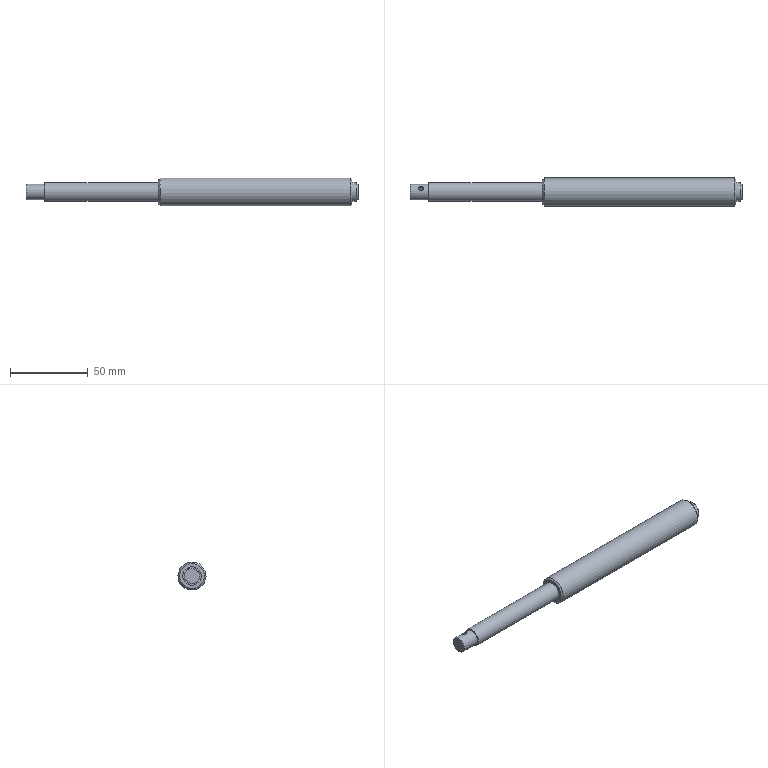Component | NX | SHAFT | 1 solid | 22 faces | volume 40331 mm3 | plane 10 | cylinder 8 | cone 3 | torus 1 | commonest cylinder face diameters 12 x2 5 x2 8 x1 3 x1 10 x1 18 x1